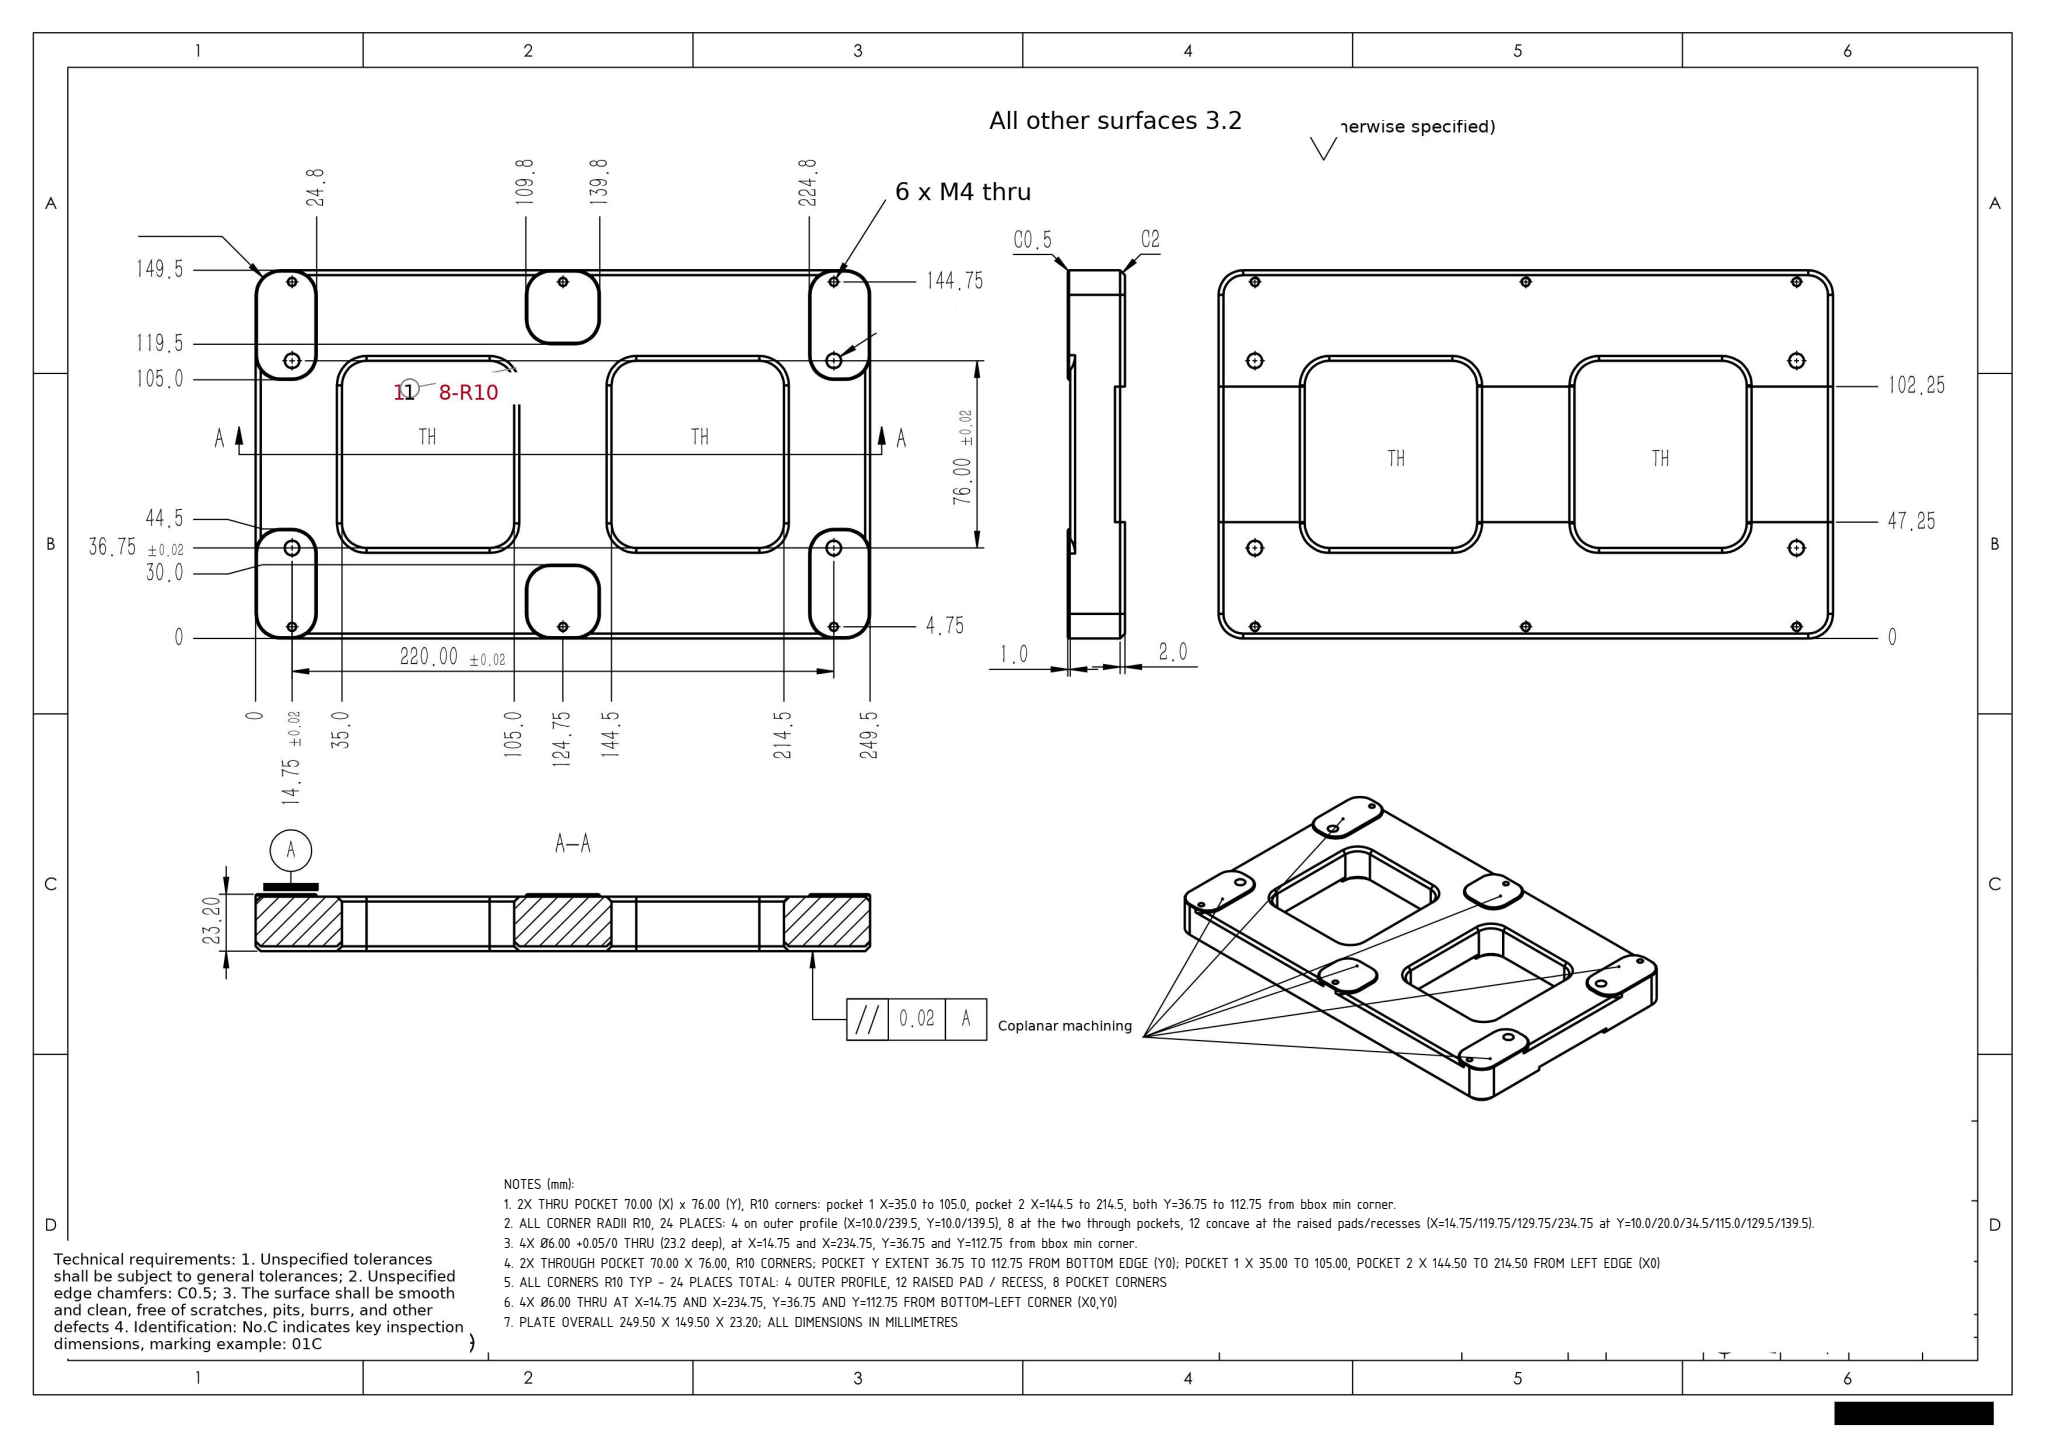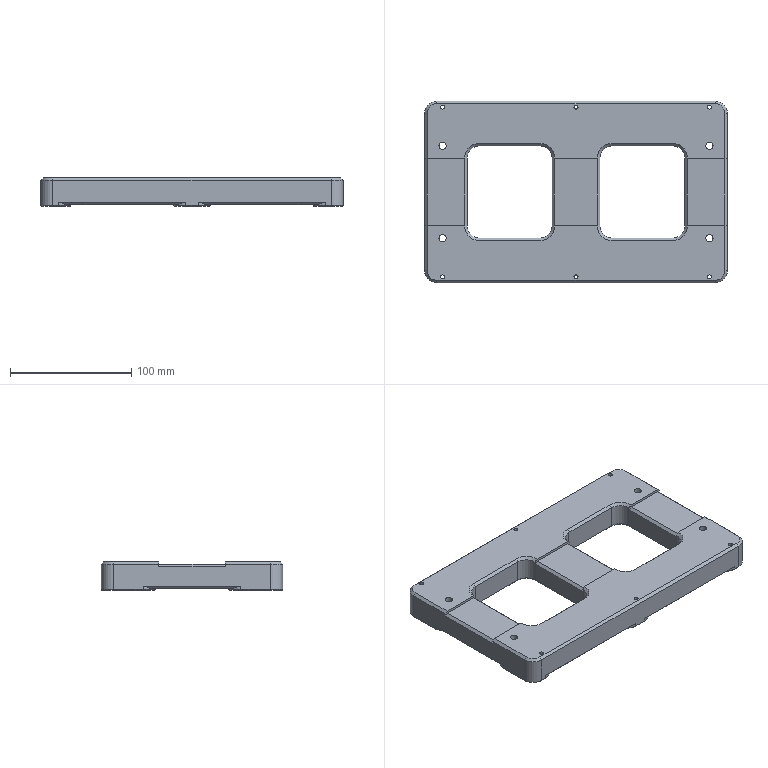Part | SolidWorks | mm | 1 solid | 202 faces | box 249.5 x 149.5 x 23.2 mm | volume 578640 mm3 | plane 106 | cylinder 52 | cone 44 | commonest cylinder face diameters 20 x32 3.3 x12 6 x8
Drawing notes:
2X THRU POCKET 70.00 (X) x 76.00 (Y), R10 corners: pocket 1 X=35.0 to 105.0, pocket 2 X=144.5 to 214.5, both Y=36.75 to 112.75 from bbox min corner. | from the solid: axis_planes x=35.0,105.0,144.5,214.5 and y=36.75,112.75; dia20 z-cylinders at (45,46.75),(95,46.75),(45,102.75),(95,102.75),(154.5,46.75),(204.5,46.75),(154.5,102.75),(204.5,102.75) length 18.2 (R10 pocket corners)
ALL CORNER RADII R10, 24 PLACES: 4 on outer profile (X=10.0/239.5, Y=10.0/139.5), 8 at the two through pockets, 12 concave at the raised pads/recesses (X=14.75/119.75/129.75/234.75 at Y=10.0/20.0/34.5/115.0/129.5/139.5). | from the solid: dia20 z-cylinders list (all R10): corner cylinders at (10,10),(10,139.5),(239.5,10),(239.5,139.5) length 20.7; 8 pocket-corner cylinders length 18.2; 12 pad/recess cylinders length 2.5/0.5
4X Ø6.00 +0.05/0 THRU (23.2 deep), at X=14.75 and X=234.75, Y=36.75 and Y=112.75 from bbox min corner. | from the solid: cylinders dia 6.0, axis z, positions (14.75,36.75),(14.75,112.75),(234.75,36.75),(234.75,112.75), length 23.2
2X THROUGH POCKET 70.00 X 76.00, R10 CORNERS; POCKET Y EXTENT 36.75 TO 112.75 FROM BOTTOM EDGE (Y0); POCKET 1 X 35.00 TO 105.00, POCKET 2 X 144.50 TO 214.50 FROM LEFT EDGE (X0) | from the solid: axis_planes x=35.0/105.0/144.5/214.5 and y=36.75/112.75; pocket corner cylinders dia 20 at (45,46.75),(95,102.75),(154.5,46.75),(204.5,102.75)
ALL CORNERS R10 TYP - 24 PLACES TOTAL: 4 OUTER PROFILE, 12 RAISED PAD / RECESS, 8 POCKET CORNERS | from the solid: cylinders dia 20.0 (R10) axis z, 24 instances incl. corner pads at (10,10),(10,139.5),(239.5,10),(239.5,139.5) and pocket corners
4X Ø6.00 THRU AT X=14.75 AND X=234.75, Y=36.75 AND Y=112.75 FROM BOTTOM-LEFT CORNER (X0,Y0) | from the solid: cylinders [6.0,z,(14.75,36.75)],(14.75,112.75),(234.75,36.75),(234.75,112.75), length 23.2 = full thickness
PLATE OVERALL 249.50 X 149.50 X 23.20; ALL DIMENSIONS IN MILLIMETRES | from the solid: bbox_xyz [249.5,149.5,23.2]
build123d program:
from build123d import *

# Parameters (mm, degrees)
SKETCH1_W           = 249.5
SKETCH1_H           = 149.5
BOSS_EXTRUDE1_DEPTH = 11.6
SKETCH2_R           = 3
CUT_EXTRUDE1_DEPTH  = 148.27
M4_TAPPED_HOLE1_D   = 3.3
SKETCH5_W           = 1
SKETCH5_H           = 60.5
CUT_EXTRUDE2_DEPTH  = 261.715
SKETCH6_W           = 85
SKETCH6_H           = 1
CUT_EXTRUDE3_DEPTH  = 196.057
SKETCH7_W           = 30
SKETCH7_H           = 14.5
CUT_EXTRUDE4_DEPTH  = 1
SKETCH8_W           = 70
SKETCH8_H           = 76
CUT_EXTRUDE5_DEPTH  = 148.115
SKETCH9_W           = 2
SKETCH9_H           = 55
CUT_EXTRUDE6_DEPTH  = 261.715
FILLET1_R           = 10
CHAMFER1_SIZE       = 0.5
CHAMFER2_SIZE       = 2


with BuildPart() as part:
    # Sketch1 → Boss-Extrude1 (new, symmetric)
    with BuildSketch(Plane.XY):
        Rectangle(SKETCH1_W, SKETCH1_H)
    extrude(amount=BOSS_EXTRUDE1_DEPTH, both=True)

    # Sketch2 → Cut-Extrude1 (cut, through all)
    with BuildSketch(Plane(origin=(0, 0, -11.6), x_dir=(-1, 0, 0), z_dir=(0, 0, -1))):
        with Locations((-110, 38)):
            Circle(SKETCH2_R)
        with Locations(Location((-110, -38, 0), (0, 0, 180))):
            Circle(SKETCH2_R)
        with Locations((110, -38)):
            Circle(SKETCH2_R)
        with Locations(Location((110, 38, 0), (0, 0, 180))):
            Circle(SKETCH2_R)
    extrude(amount=-CUT_EXTRUDE1_DEPTH, mode=Mode.SUBTRACT)

    # M4 Tapped Hole1 (through all)
    with Locations(Plane.XY.offset(11.6)):
        with Locations((-110, 70), (110, 70), (110, -70), (-110, -70), (0, 70), (0, -70)):
            Hole(M4_TAPPED_HOLE1_D / 2)

    # Sketch5 → Cut-Extrude2 (cut, through all)
    with BuildSketch(Plane(origin=(124.75, 0, 0), x_dir=(0, 0, -1), z_dir=(1, 0, 0))):
        with Locations((11.1, 0)):
            Rectangle(SKETCH5_W, SKETCH5_H)
    extrude(amount=-CUT_EXTRUDE2_DEPTH, mode=Mode.SUBTRACT)

    # Sketch6 → Cut-Extrude3 (cut, through all)
    with BuildSketch(Plane.XZ.offset(74.75)):
        with Locations((57.5, -11.1)):
            Rectangle(SKETCH6_W, SKETCH6_H)
        with Locations((-57.5, -11.1)):
            Rectangle(SKETCH6_W, SKETCH6_H)
    extrude(amount=-CUT_EXTRUDE3_DEPTH, mode=Mode.SUBTRACT)

    # Sketch7 → Cut-Extrude4 (cut)
    with BuildSketch(Plane(origin=(0, 0, -11.6), x_dir=(-1, 0, 0), z_dir=(0, 0, -1))):
        with Locations((0, 37.5)):
            Rectangle(SKETCH7_W, SKETCH7_H)
        with Locations((0, -37.5)):
            Rectangle(SKETCH7_W, SKETCH7_H)
    extrude(amount=-CUT_EXTRUDE4_DEPTH, mode=Mode.SUBTRACT)

    # Sketch8 → Cut-Extrude5 (cut, through all)
    with BuildSketch(Plane(origin=(0, 0, -10.6), x_dir=(-1, 0, 0), z_dir=(0, 0, -1))):
        with Locations((54.75, 0)):
            Rectangle(SKETCH8_W, SKETCH8_H)
        with Locations((-54.75, 0)):
            Rectangle(SKETCH8_W, SKETCH8_H)
    extrude(amount=-CUT_EXTRUDE5_DEPTH, mode=Mode.SUBTRACT)

    # Sketch9 → Cut-Extrude6 (cut, through all)
    with BuildSketch(Plane.ZY.offset(124.75)):
        with Locations((10.6, 0)):
            Rectangle(SKETCH9_W, SKETCH9_H)
    extrude(amount=-CUT_EXTRUDE6_DEPTH, mode=Mode.SUBTRACT)

    # Fillet1
    fillet1_edges = [part.edges().sort_by_distance(p)[0] for p in [
        (-100, 30.25, -11.1),
        (-100, 74.75, -11.1),
        (-100, -30.25, -11.1),
        (-15, 74.75, -11.1),
        (-100, -74.75, -11.1),
        (-15, -74.75, -11.1),
        (15, 44.75, -11.1),
        (-15, 44.75, -11.1),
        (-15, -44.75, -11.1),
        (15, -44.75, -11.1),
        (-19.75, -38, 0.5),
        (-19.75, 38, 0.5),
        (-89.75, 38, 0.5),
        (-89.75, -38, 0.5),
        (89.75, -38, 0.5),
        (89.75, 38, 0.5),
        (19.75, 38, 0.5),
        (19.75, -38, 0.5),
        (-124.75, 30.25, -11.1),
        (-124.75, -30.25, -11.1),
        (124.75, -30.25, -11.1),
        (124.75, 30.25, -11.1),
        (124.75, -74.75, 0),
        (-124.75, -74.75, 0),
        (-124.75, 74.75, 0),
        (124.75, 74.75, 0),
        (100, -30.25, -11.1),
        (15, 74.75, -11.1),
        (100, 30.25, -11.1),
        (100, 74.75, -11.1),
        (15, -74.75, -11.1),
        (100, -74.75, -11.1),
    ]]
    fillet(fillet1_edges, radius=FILLET1_R)

    # Chamfer1
    chamfer1_edges = [part.edges().sort_by_distance(p)[0] for p in [
        (0, -44.75, -11.6),
        (15, -59.75, -11.6),
        (0, -74.75, -11.6),
        (-15, -59.75, -11.6),
        (-12.071, -71.821, -11.6),
        (12.071, -71.821, -11.6),
        (-12.071, -47.679, -11.6),
        (12.071, -47.679, -11.6),
        (15, 59.75, -11.6),
        (0, 44.75, -11.6),
        (-15, 59.75, -11.6),
        (0, 74.75, -11.6),
        (-12.071, 71.821, -11.6),
        (12.071, 71.821, -11.6),
        (-12.071, 47.679, -11.6),
        (12.071, 47.679, -11.6),
        (-124.75, 52.5, -11.6),
        (-124.75, -52.5, -11.6),
        (-100, -52.5, -11.6),
        (-112.375, -74.75, -11.6),
        (-112.375, -30.25, -11.6),
        (-121.821, -71.821, -11.6),
        (-102.929, -33.179, -11.6),
        (-102.929, -71.821, -11.6),
        (-121.821, -33.179, -11.6),
        (112.375, -74.75, -11.6),
        (-112.375, 30.25, -11.6),
        (-100, 52.5, -11.6),
        (-112.375, 74.75, -11.6),
        (-121.821, 71.821, -11.6),
        (-102.929, 33.179, -11.6),
        (-102.929, 71.821, -11.6),
        (-121.821, 33.179, -11.6),
        (112.375, 74.75, -11.6),
        (112.375, -30.25, -11.6),
        (100, -52.5, -11.6),
        (124.75, -52.5, -11.6),
        (121.821, -71.821, -11.6),
        (102.929, -33.179, -11.6),
        (102.929, -71.821, -11.6),
        (121.821, -33.179, -11.6),
        (124.75, 52.5, -11.6),
        (100, 52.5, -11.6),
        (112.375, 30.25, -11.6),
        (121.821, 71.821, -11.6),
        (102.929, 33.179, -11.6),
        (121.821, 33.179, -11.6),
        (102.929, 71.821, -11.6),
    ]]
    chamfer(chamfer1_edges, length=CHAMFER1_SIZE)

    # Chamfer2
    chamfer2_edges = [part.edges().sort_by_distance(p)[0] for p in [
        (-86.821, 35.071, -10.6),
        (-89.75, 0, -10.6),
        (-86.821, -35.071, -10.6),
        (-54.75, -38, -10.6),
        (-22.679, -35.071, -10.6),
        (-19.75, 0, -10.6),
        (-22.679, 35.071, -10.6),
        (-54.75, 38, -10.6),
        (19.75, 0, -10.6),
        (22.679, -35.071, -10.6),
        (54.75, -38, -10.6),
        (86.821, -35.071, -10.6),
        (89.75, 0, -10.6),
        (86.821, 35.071, -10.6),
        (54.75, 38, -10.6),
        (22.679, 35.071, -10.6),
        (22.679, 35.071, 11.6),
        (19.75, -27.75, 11.6),
        (19.75, 27.75, 11.6),
        (22.679, -35.071, 11.6),
        (54.75, -38, 11.6),
        (86.821, -35.071, 11.6),
        (89.75, 27.75, 11.6),
        (89.75, -27.75, 11.6),
        (86.821, 35.071, 11.6),
        (54.75, 38, 11.6),
        (-86.821, -35.071, 11.6),
        (-89.75, 27.75, 11.6),
        (-89.75, -27.75, 11.6),
        (-86.821, 35.071, 11.6),
        (-54.75, 38, 11.6),
        (-22.679, 35.071, 11.6),
        (-19.75, 27.75, 11.6),
        (-19.75, -27.75, 11.6),
        (-22.679, -35.071, 11.6),
        (-54.75, -38, 11.6),
        (-124.75, 0, -10.6),
        (-57.5, 74.75, -10.6),
        (57.5, 74.75, -10.6),
        (57.5, -74.75, -10.6),
        (-121.821, -71.821, 11.6),
        (-121.821, 71.821, 11.6),
        (0, 74.75, 11.6),
        (121.821, 71.821, 11.6),
        (0, -74.75, 11.6),
        (121.821, -71.821, 11.6),
        (124.75, 46.125, 11.6),
        (124.75, -46.125, 11.6),
        (124.75, 0, -10.6),
        (-57.5, -74.75, -10.6),
        (-124.75, -46.125, 11.6),
        (-124.75, 46.125, 11.6),
        (89.75, 0, 9.6),
        (19.75, 0, 9.6),
        (-19.75, 0, 9.6),
        (-89.75, 0, 9.6),
        (-124.75, 0, 9.6),
        (124.75, 0, 9.6),
    ]]
    chamfer(chamfer2_edges, length=CHAMFER2_SIZE)


solid = part.part